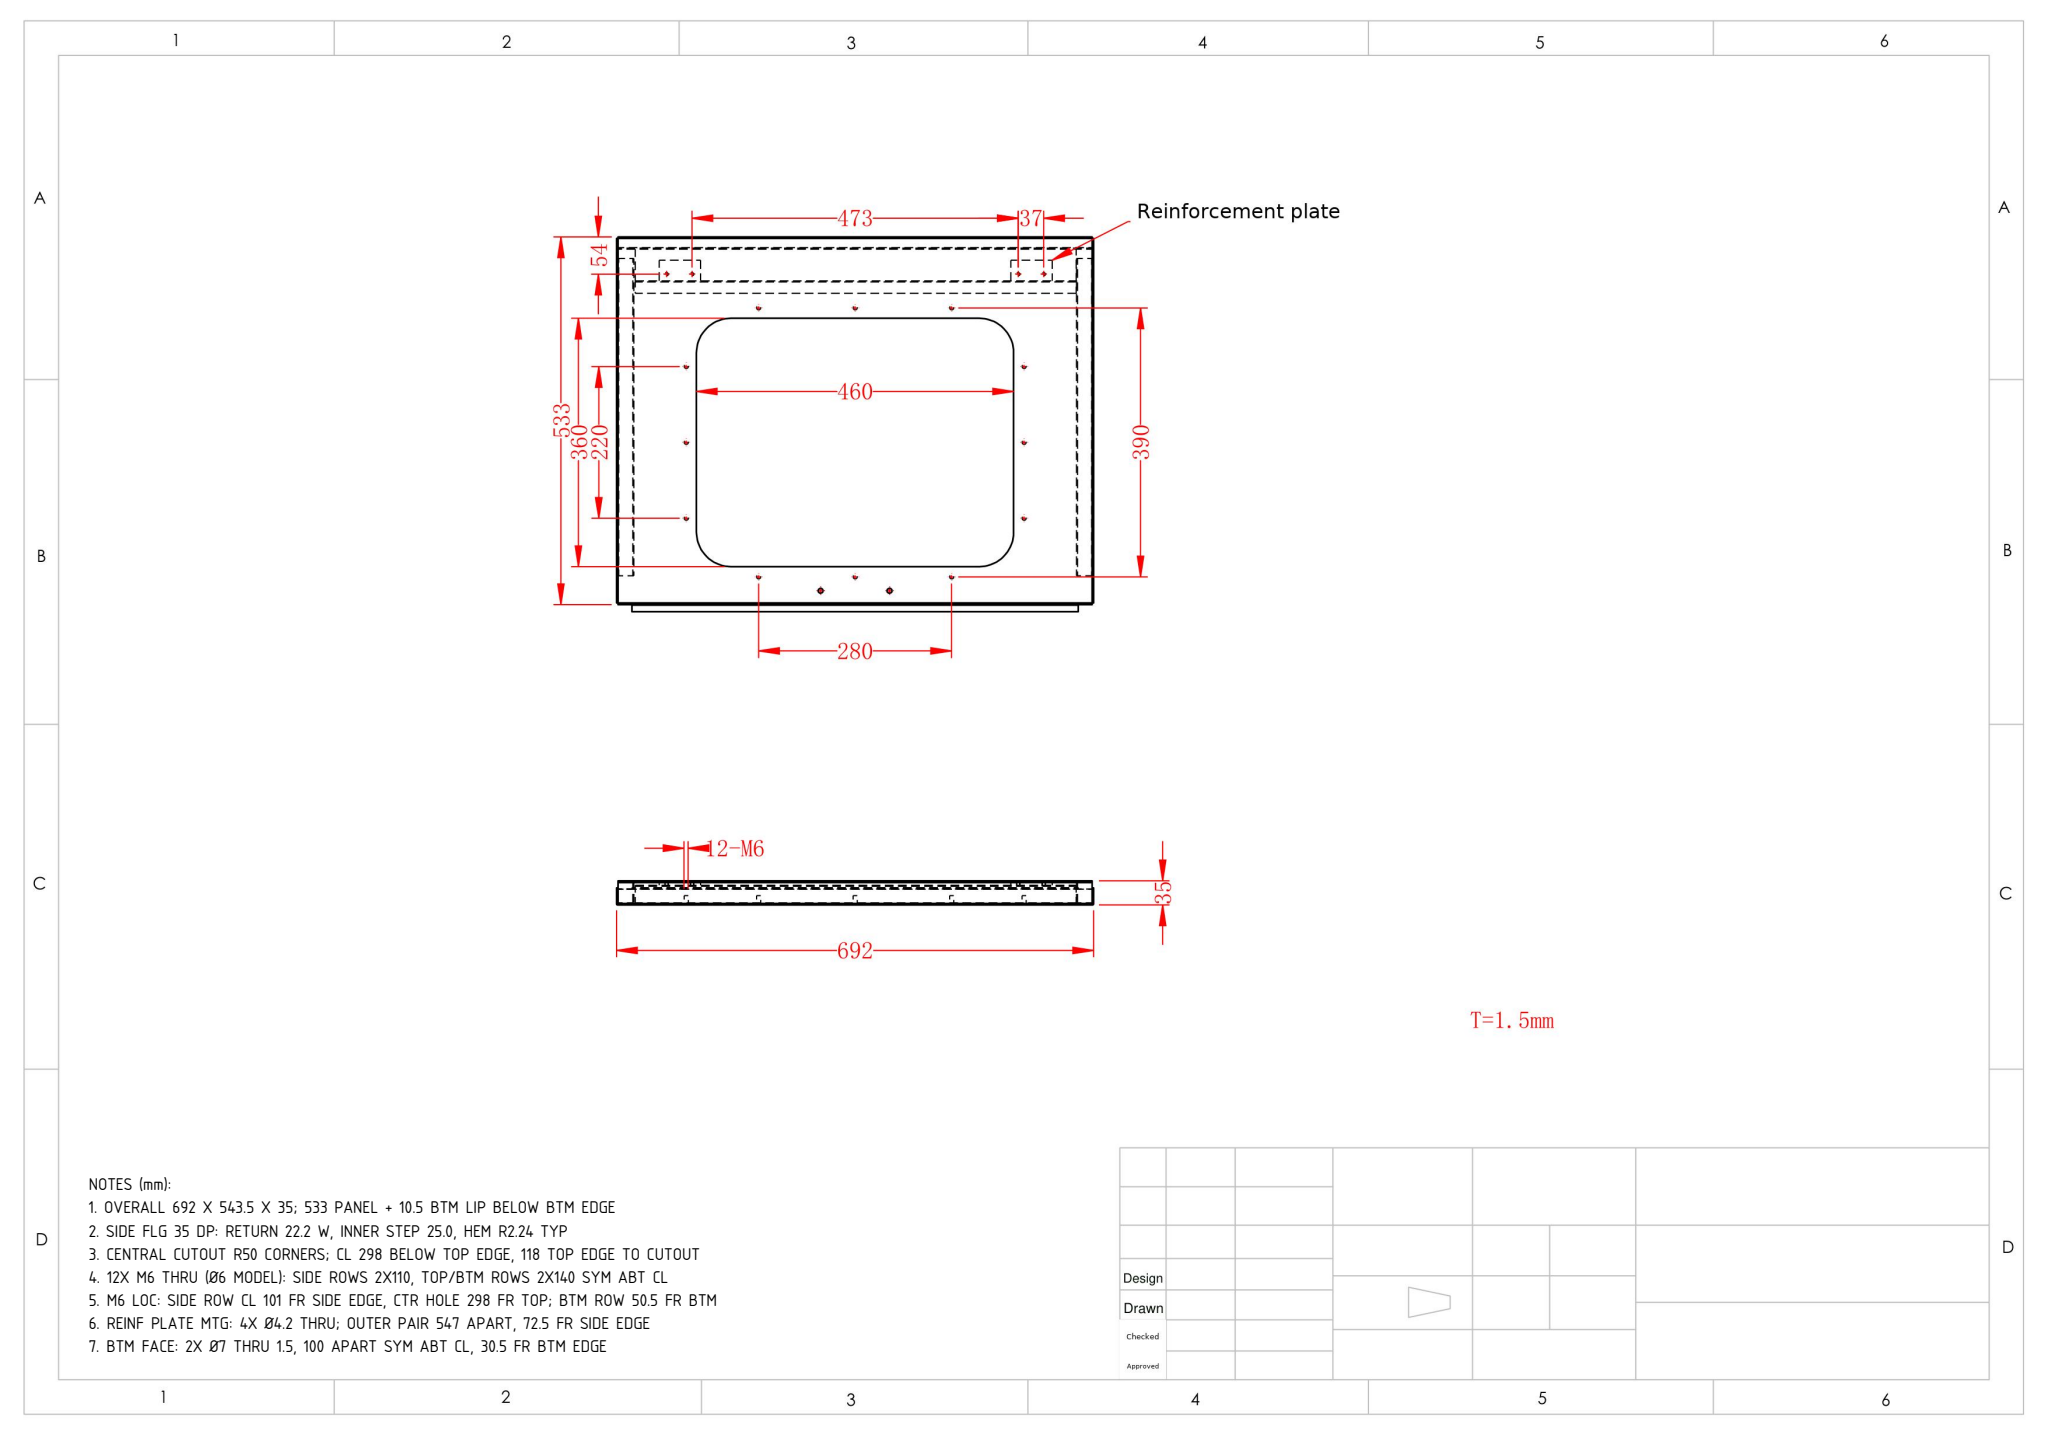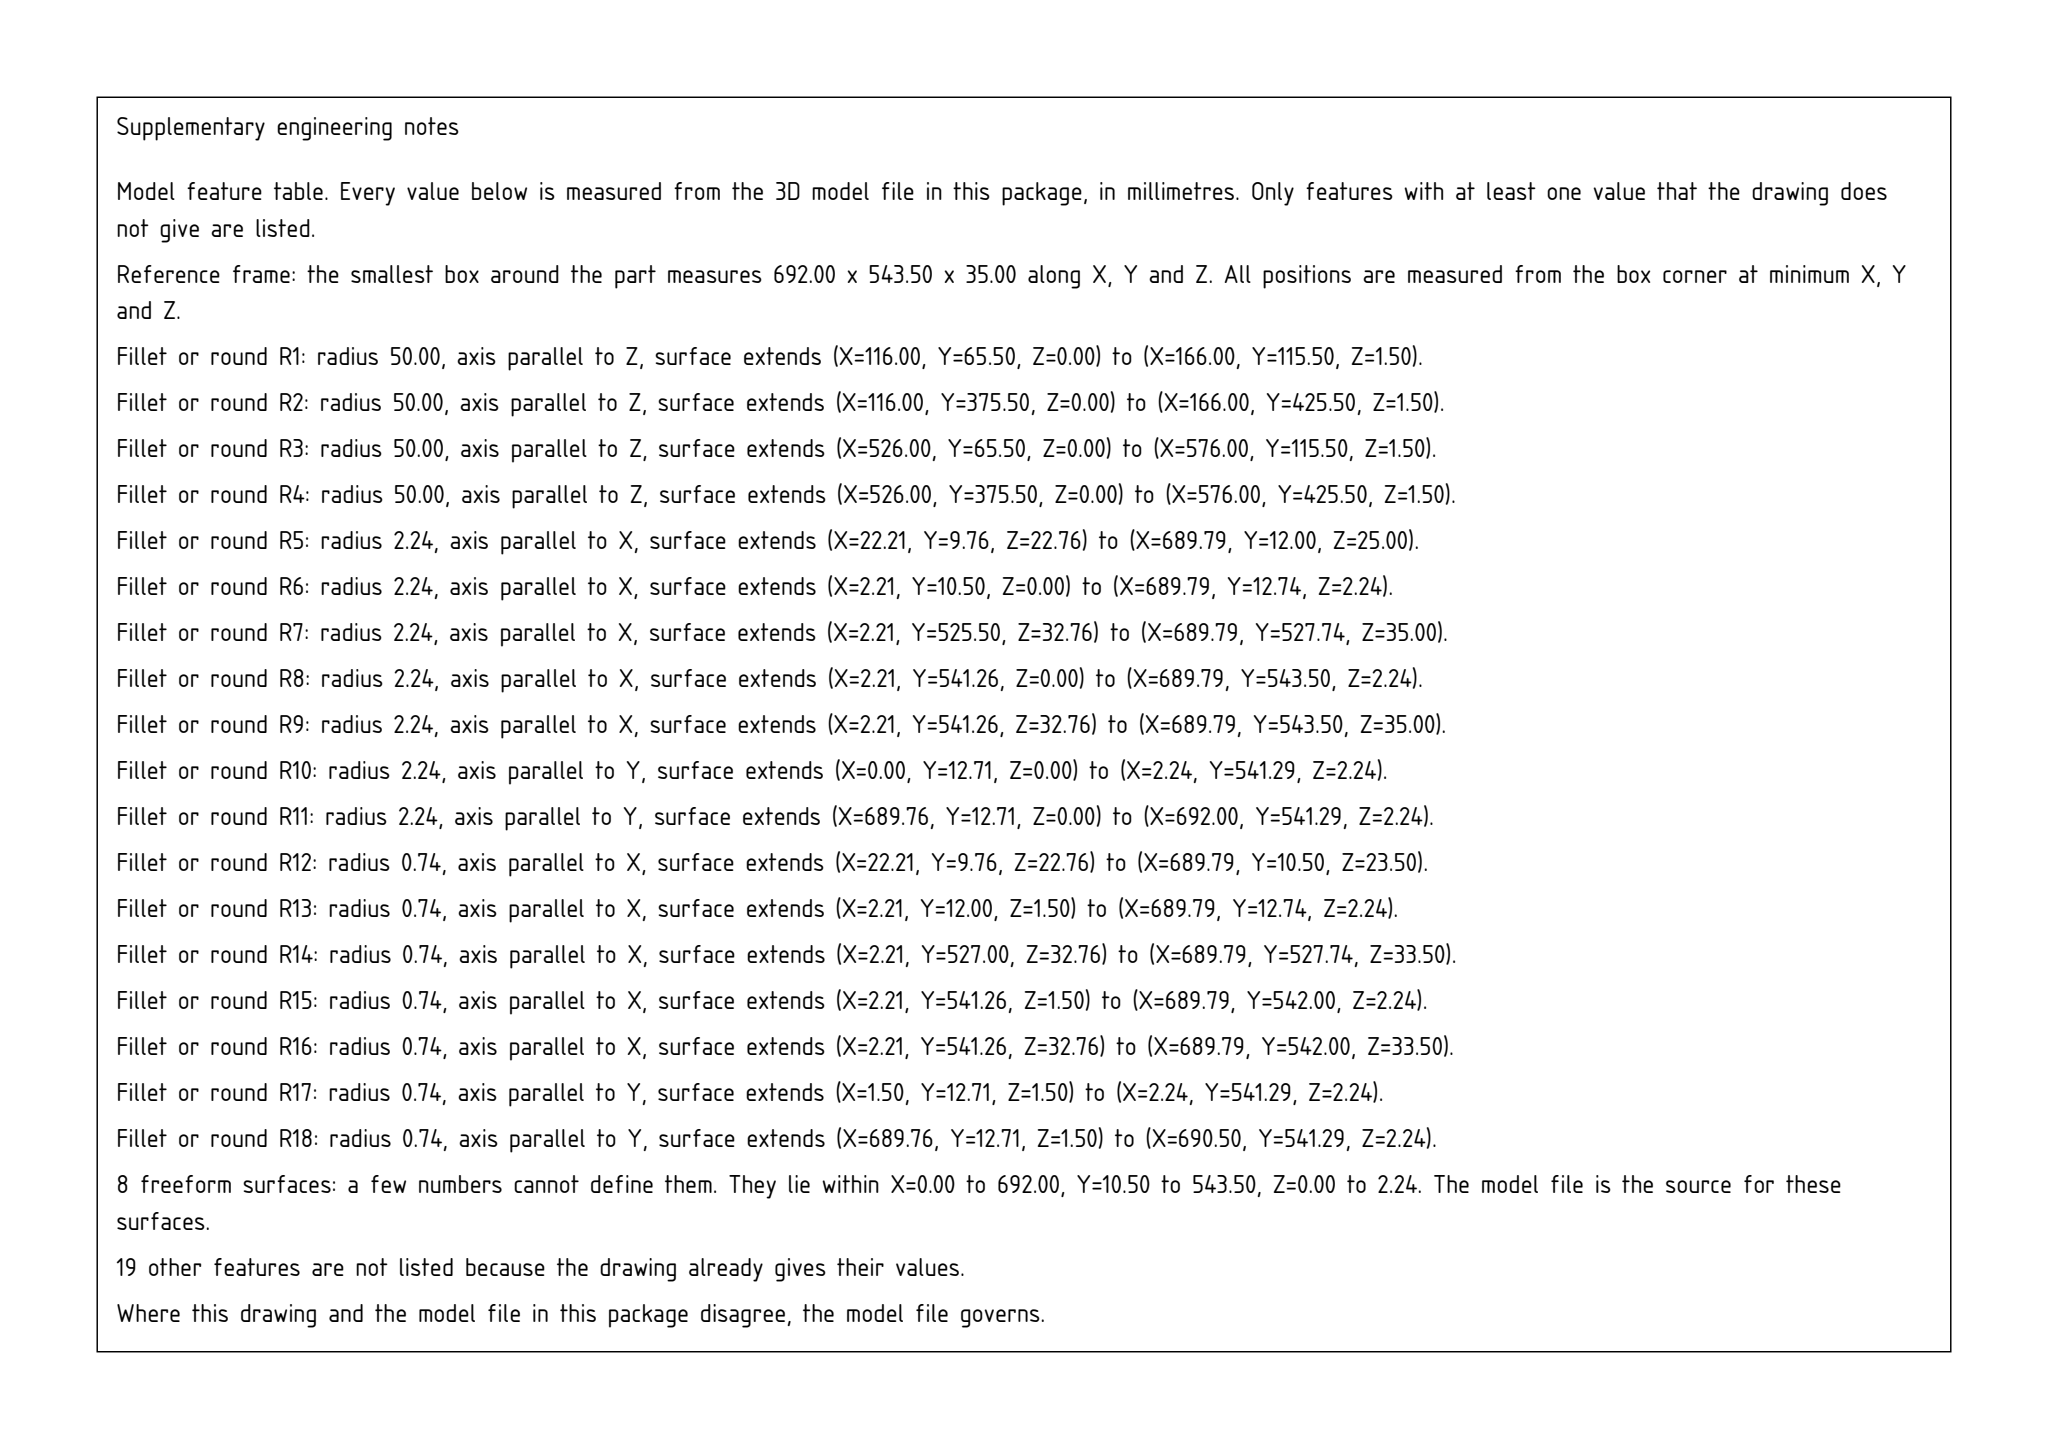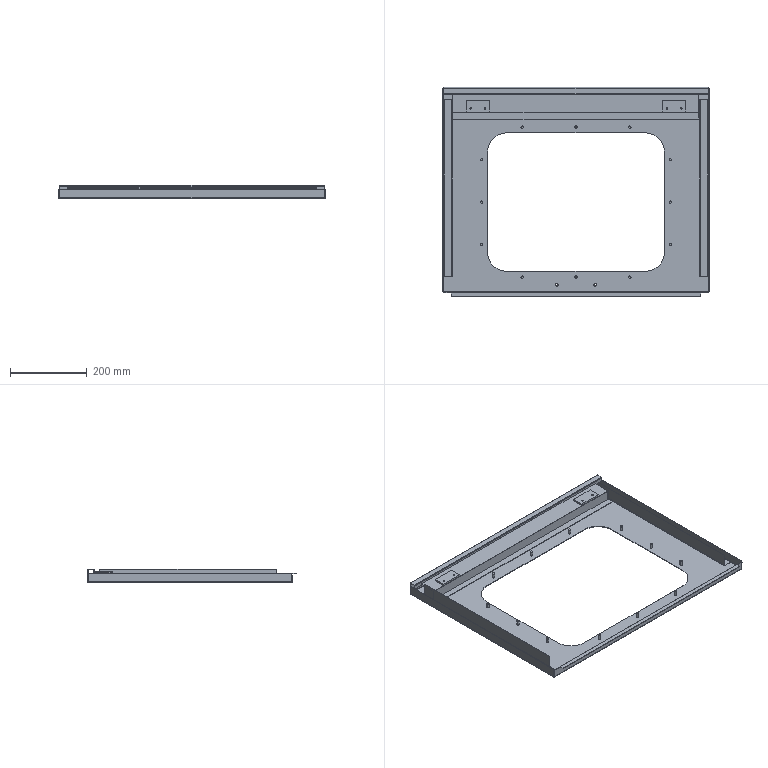Part | SolidWorks | mm | 1 solid | 153 faces | box 692 x 543.5 x 35 mm | volume 617946 mm3 | plane 91 | cylinder 54 | spline 8 | commonest cylinder face diameters 6 x24 4.2 x8 4.473 x7 1.473 x7 7 x4 100 x4
Drawing notes:
OVERALL 692 X 543.5 X 35; 533 PANEL + 10.5 BTM LIP BELOW BTM EDGE | from the solid: bbox 692.03 x 543.515 x 35.015; y-planes 0 / 10.5 / 543.5 => 543.5-10.5=533
SIDE FLG 35 DP: RETURN 22.2 W, INNER STEP 25.0, HEM R2.24 TYP | from the solid: x-planes 0.02/1.52/2.22/3.02/22.22/23.52/25.02/25.52 mirrored at 692.02; Ø4.473 hem cyls
CENTRAL CUTOUT R50 CORNERS; CL 298 BELOW TOP EDGE, 118 TOP EDGE TO CUTOUT | from the solid: 4X Ø100 z-cyls L=1.5 at x=166.02/526.02, y=115.5/375.5 -> cutout y 65.5..425.5, CL 245.5
12X M6 THRU (Ø6 MODEL): SIDE ROWS 2X110, TOP/BTM ROWS 2X140 SYM ABT CL | from the solid: Ø6 z-cyls L=12: x=101.02/591.02 at y=135.5/245.5/355.5; x=206.02/346.02/486.02 rows
M6 LOC: SIDE ROW CL 101 FR SIDE EDGE, CTR HOLE 298 FR TOP; BTM ROW 50.5 FR BTM | from the solid: x=101.02 & 692.03-591.02=101.01; 543.5-245.5=298; y=50.5, top row y=440.5
REINF PLATE MTG: 4X Ø4.2 THRU; OUTER PAIR 547 APART, 72.5 FR SIDE EDGE | from the solid: Ø4.2 z-holes x=72.52/109.52/582.52/619.52 at y=489.5; 619.52-72.52=547; CL 346.02
BTM FACE: 2X Ø7 THRU 1.5, 100 APART SYM ABT CL, 30.5 FR BTM EDGE | from the solid: Ø7 z-holes L=1.5 at x=296.02 & 396.02 (ctr 346.02), y=30.5